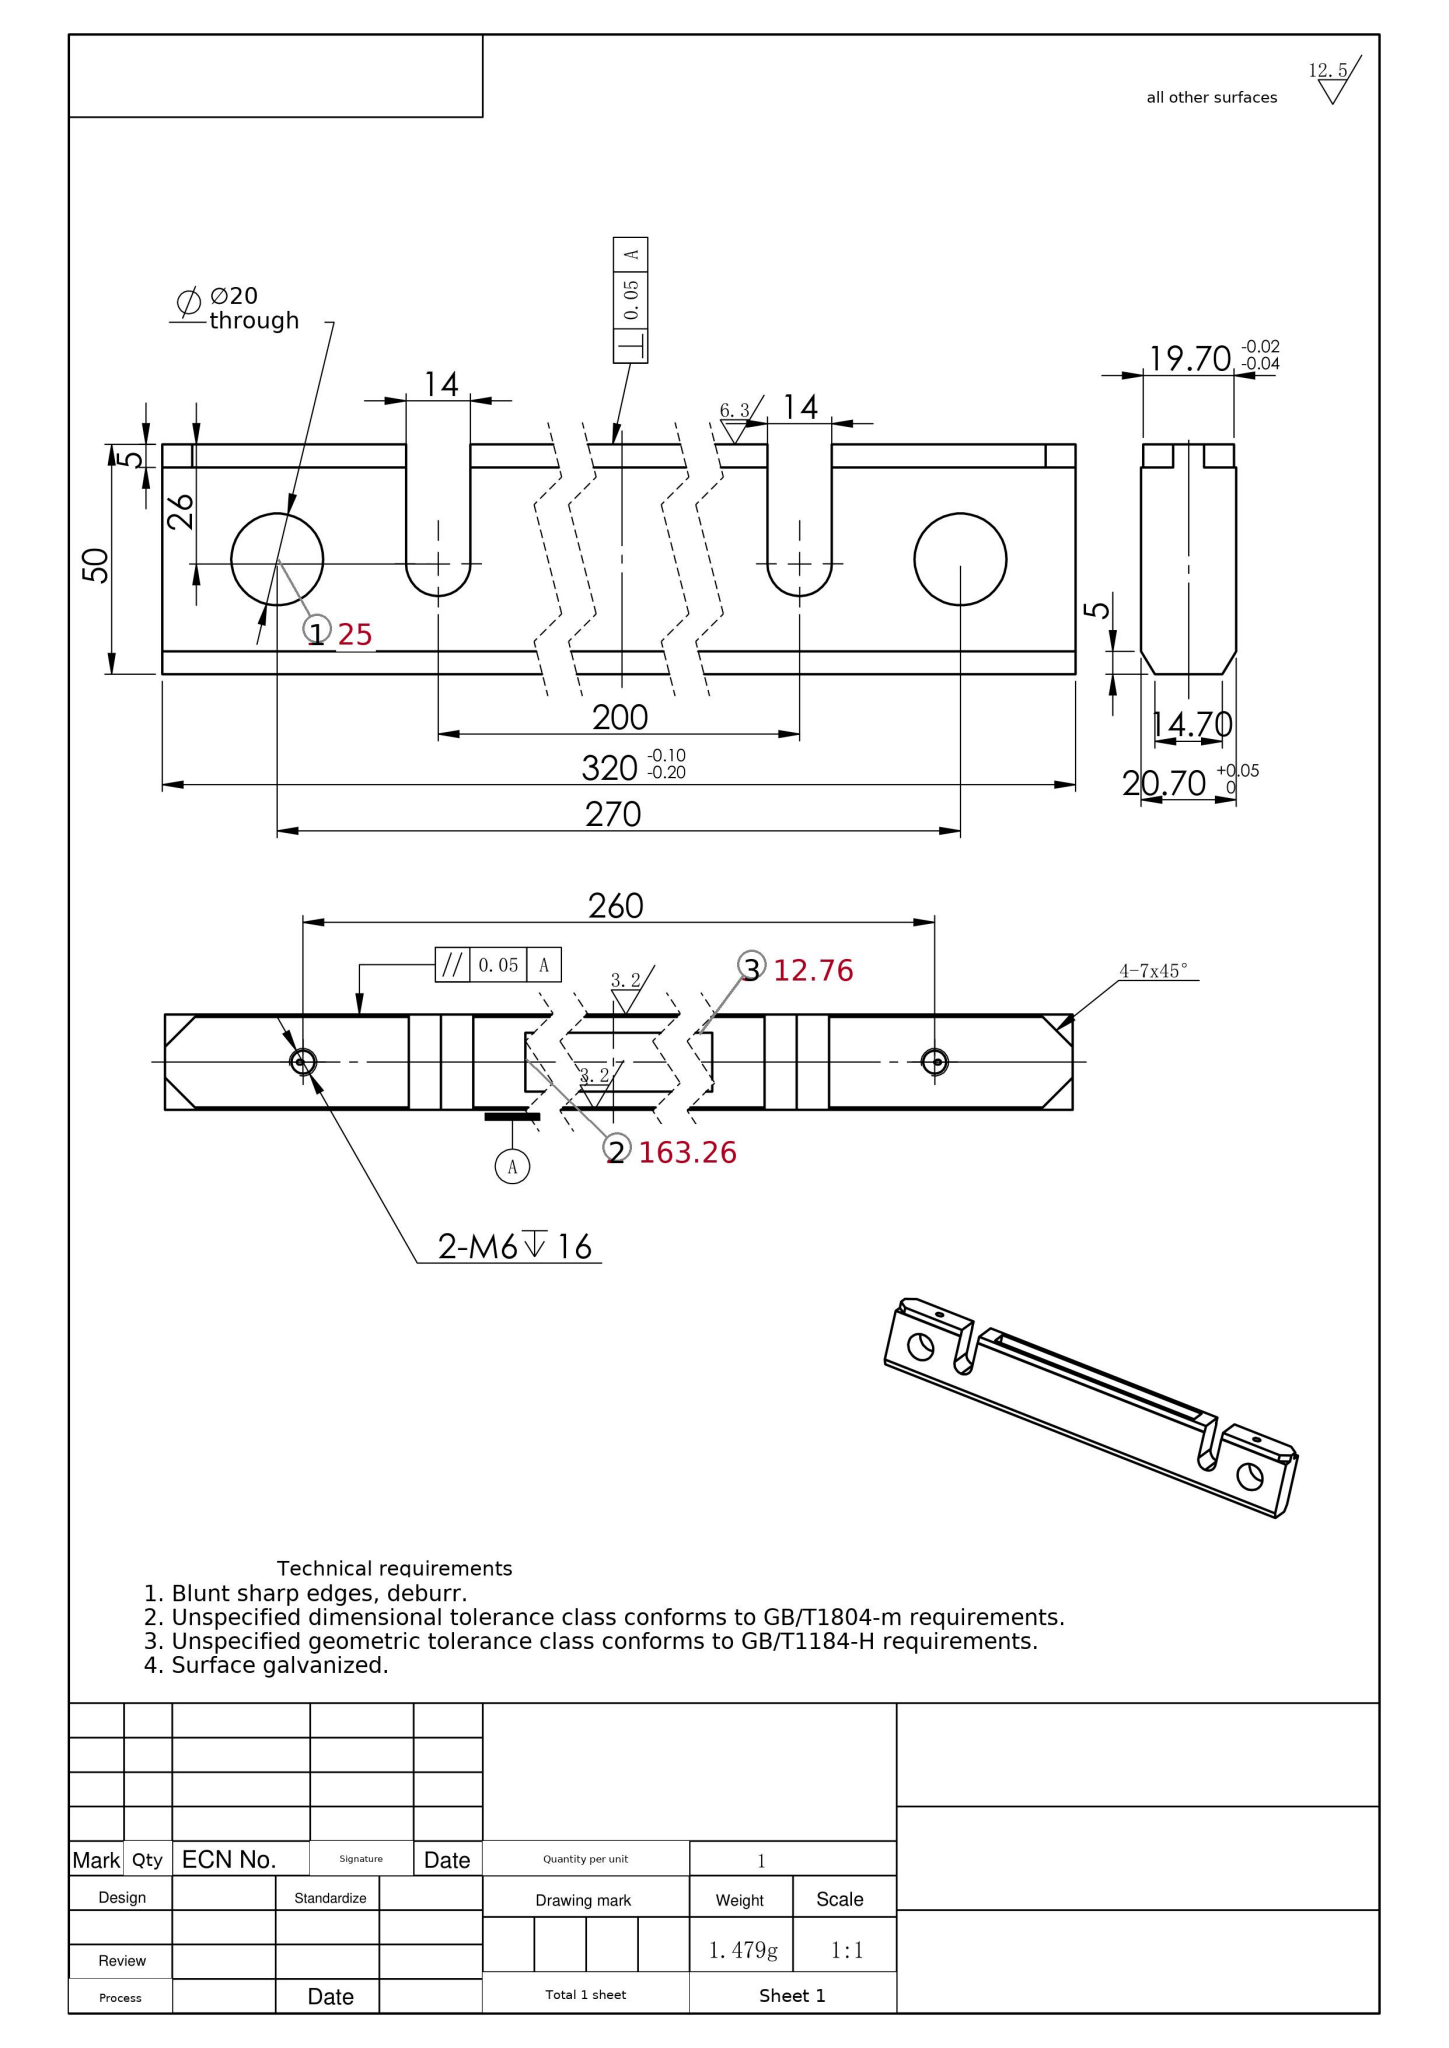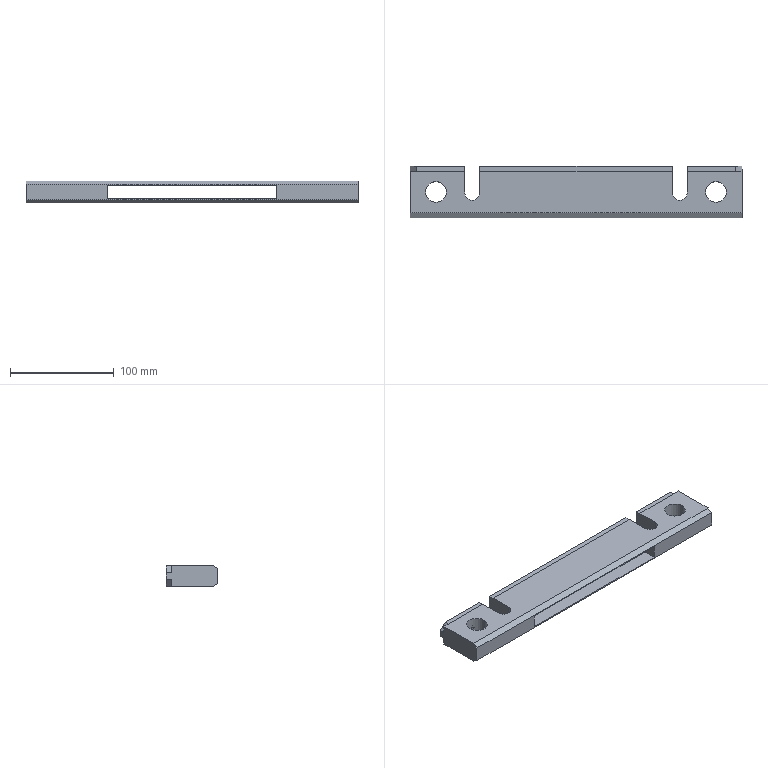Part | SolidWorks | mm | 1 solid | 50 faces | box 320 x 50 x 20.7 mm | volume 188452 mm3 | plane 34 | cylinder 12 | cone 4 | commonest cylinder face diameters 20 x4 5 x4 14 x4